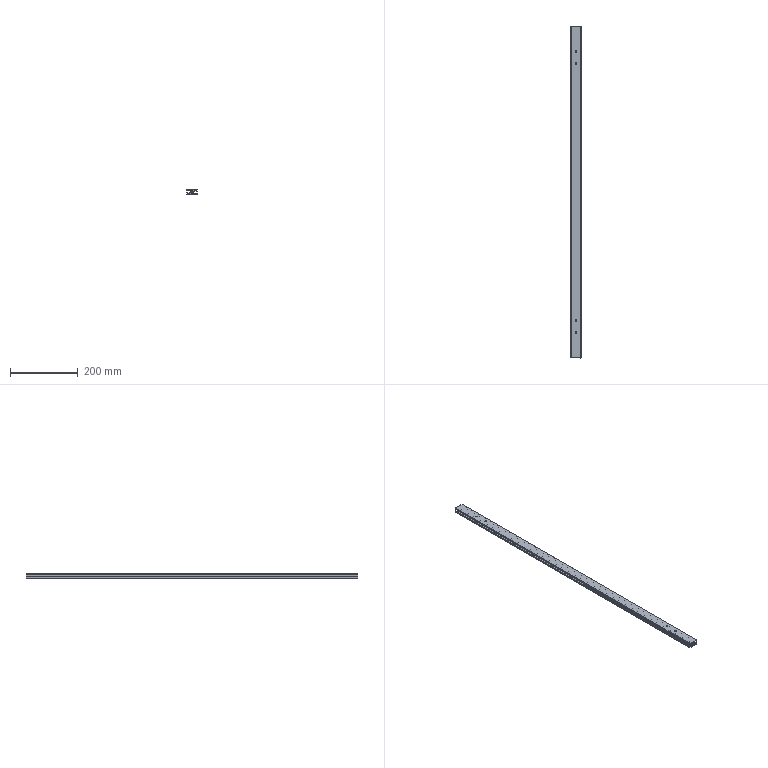Component | SolidWorks | 2012MB0201-1_ASideDoor-1-1_A3001-3 | 1 solid | 66 faces | box 30.3 x 982 x 15.67 mm | volume 237570 mm3 | cylinder 34 | plane 32 | commonest cylinder face diameters 5 x26 6 x4 2 x4
build123d program:
from build123d import *

# Parameters (mm, degrees)
SKETCH1_2_W                 = 30
SKETCH1_2_H                 = 15
BOSS_EXTRUDE1_DEPTH         = 982
SKETCH2_2_R                 = 2.5
CUT_EXTRUDE1_DEPTH          = 983.143
FILLET1_R                   = 1
M6_TAPPED_HOLE1_D           = 5
SKETCH1_R                   = 3
M6_THREADED_END_HOLE1_DEPTH = 13
M6_START                    = -13
SKETCH2_R                   = 3
M6_THREADED_END_HOLE2_DEPTH = 13


with BuildPart() as part:
    # Sketch1_2 → Boss-Extrude1 (new body)
    with BuildSketch(Plane(origin=(0, 0, 0), x_dir=(1, 0, 0), z_dir=(0, 1, 0))):
        Rectangle(SKETCH1_2_W, SKETCH1_2_H)
    extrude(amount=BOSS_EXTRUDE1_DEPTH)

    # Sketch2_2 → Cut-Extrude1 (cut, through all)
    with BuildSketch(Plane.XZ):
        with Locations(Location((0, 0, 0), (0, 0, 270))):
            Circle(SKETCH2_2_R)
        Polygon((15, -3.25), (12.6, -3.25), (12.6, -5.3), (6.6, -5.3), (6.6, -2.926), (4.2, -2.926), (4.2, 2.926), (6.6, 2.926), (6.6, 5.3), (12.6, 5.3), (12.6, 3.25), (15, 3.25), align=None)
        Polygon((-6.6, -2.926), (-4.2, -2.926), (-4.2, 2.926), (-6.6, 2.926), (-6.6, 5.3), (-12.6, 5.3), (-12.6, 3.25), (-15, 3.25), (-15, -3.25), (-12.6, -3.25), (-12.6, -5.3), (-6.6, -5.3), align=None)
    extrude(amount=-CUT_EXTRUDE1_DEPTH, mode=Mode.SUBTRACT)

    # Fillet1
    fillet1_edges = [part.edges().sort_by_distance(p)[0] for p in [
        (15, 491, 7.5),
        (-15, 491, 7.5),
        (-15, 491, -7.5),
        (15, 491, -7.5),
    ]]
    fillet(fillet1_edges, radius=FILLET1_R)

    # M6 Tapped Hole1 (through all)
    with Locations(Plane.XY.offset(7.5)):
        with Locations((0, 907), (0, 871), (0, 111), (0, 75)):
            Hole(M6_TAPPED_HOLE1_D / 2)

    # Sketch1 → M6 Threaded End Hole1 (cut)
    with BuildSketch(Plane.XZ):
        Circle(SKETCH1_R)
    extrude(amount=-M6_THREADED_END_HOLE1_DEPTH, mode=Mode.SUBTRACT)

    # Sketch2 → M6 Threaded End Hole2 (cut)
    with BuildSketch(Plane(origin=(0, 982, 0), x_dir=(1, 0, 0), z_dir=(0, 1, 0)).offset(M6_START)):
        Circle(SKETCH2_R)
    extrude(amount=M6_THREADED_END_HOLE2_DEPTH, mode=Mode.SUBTRACT)


solid = part.part

# Placed as in the assembly
solid = solid.moved(Location((-837.925, 972.35, -189.468), (0, 1.371, -180)))